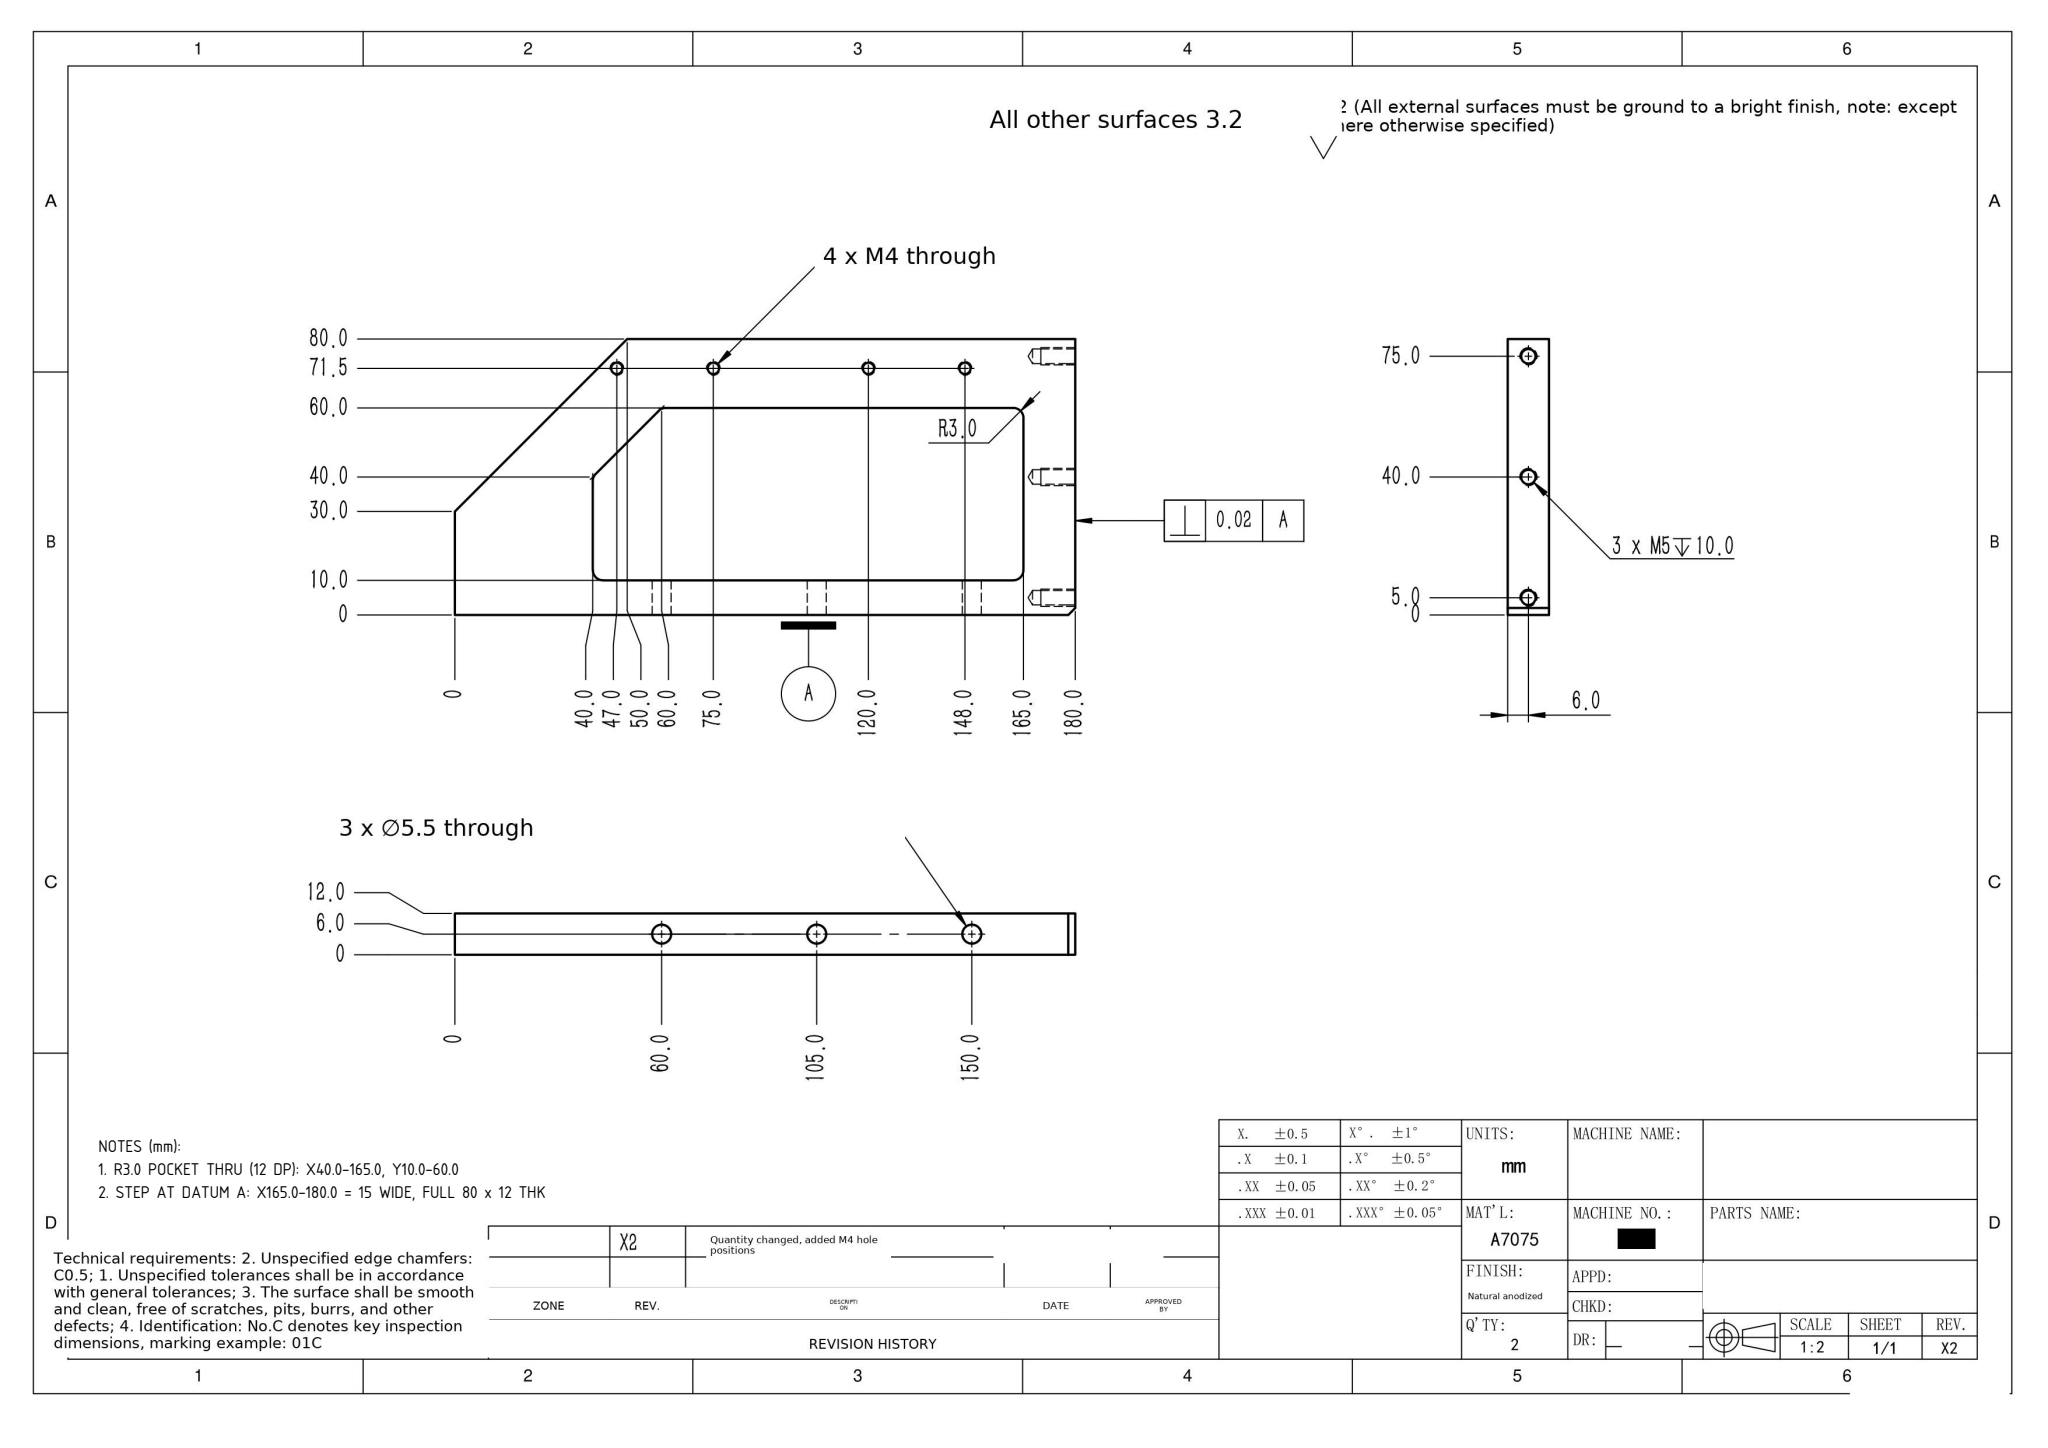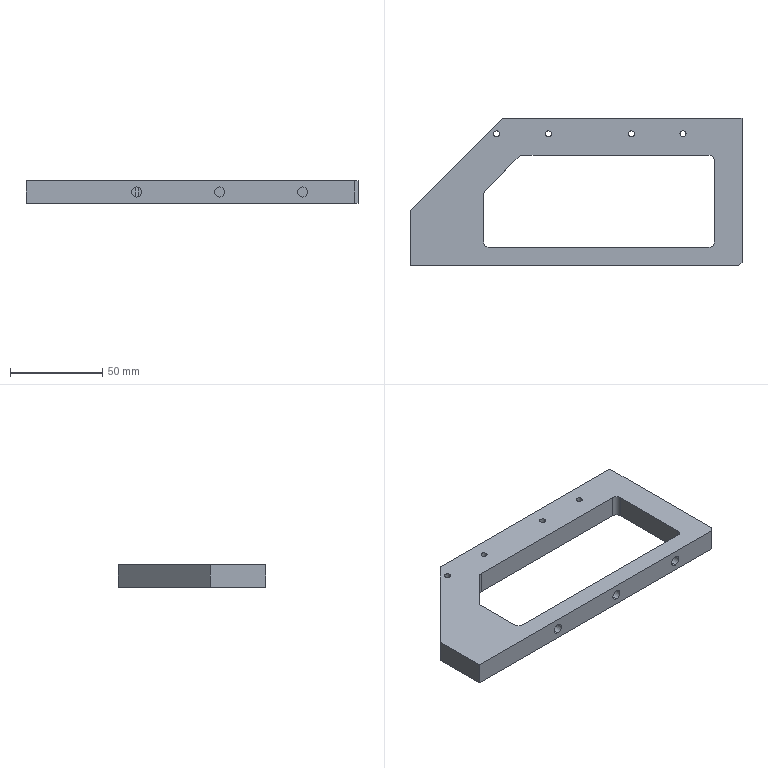Part | SolidWorks | mm | 1 solid | 44 faces | box 180 x 80 x 12 mm | volume 83594 mm3 | cylinder 25 | plane 13 | cone 6 | commonest cylinder face diameters 3.3 x8 4.2 x6 5.5 x6 6 x5
Drawing notes:
R3.0 POCKET THRU (12 DP): X40.0-165.0, Y10.0-60.0 | from the solid: Ø6.0 (R3.0) corner cyls at (43,13),(43,38.76),(61.24,57),(162,13),(162,57), len 12.0 = full thk; planes x=40/165, y=10/60
STEP AT DATUM A: X165.0-180.0 = 15 WIDE, FULL 80 x 12 THK | from the solid: axis planes x=165.0 and x=180.0; bbox 180x80x12; M5 holes (Ø4.2, x-axis) at z=6.0 enter from x=180 face
build123d program:
from build123d import *

# Parameters (mm, degrees)
SKETCH1_W             = 180
SKETCH1_H             = 80
BOSS_EXTRUDE1_DEPTH   = 6
CHAMFER1_SIZE         = 50
SKETCH2_W             = 125
SKETCH2_H             = 50
CUT_EXTRUDE1_DEPTH    = 100.217
CHAMFER2_SIZE         = 20
SKETCH3_R             = 2.75
CUT_EXTRUDE2_DEPTH    = 10
LPATTERN1_COUNT       = 3
LPATTERN1_PITCH       = 45
M5_TAPPED_HOLE1_D     = 4.2
M5_TAPPED_HOLE1_DEPTH = 12.4
M5_TAPPED_HOLE1_TIP   = 1.262
FILLET1_R             = 3
CHAMFER3_SIZE         = 2
M4_TAPPED_HOLE1_D     = 3.3


with BuildPart() as part:
    # Sketch1 → Boss-Extrude1 (new, symmetric)
    with BuildSketch(Plane.XY):
        Rectangle(SKETCH1_W, SKETCH1_H)
    extrude(amount=BOSS_EXTRUDE1_DEPTH, both=True)

    # Chamfer1
    chamfer1_edges = [part.edges().sort_by_distance(p)[0] for p in [
        (-90, 40, 0),
    ]]
    chamfer(chamfer1_edges, length=CHAMFER1_SIZE)

    # Sketch2 → Cut-Extrude1 (cut, through all)
    with BuildSketch(Plane.XY.offset(6)):
        with Locations((12.5, -5)):
            Rectangle(SKETCH2_W, SKETCH2_H)
    extrude(amount=-CUT_EXTRUDE1_DEPTH, mode=Mode.SUBTRACT)

    # Chamfer2
    chamfer2_edges = [part.edges().sort_by_distance(p)[0] for p in [
        (-50, 20, 0),
    ]]
    chamfer(chamfer2_edges, length=CHAMFER2_SIZE)

    # Sketch3 → Cut-Extrude2 (cut)
    with BuildSketch(Plane.XZ.offset(40)):
        with Locations(Location((60, 0, 0), (0, 0, 270))):
            Circle(SKETCH3_R)
    cut_extrude2 = extrude(amount=-CUT_EXTRUDE2_DEPTH, mode=Mode.SUBTRACT)

    # LPattern1: Cut-Extrude2 ×3
    with Locations(*[(-i * LPATTERN1_PITCH, 0, 0) for i in range(1, LPATTERN1_COUNT)]):
        add(cut_extrude2, mode=Mode.SUBTRACT)

    # M5 Tapped Hole1
    with Locations(Plane(origin=(90, 0, 0), x_dir=(0, 0, -1), z_dir=(1, 0, 0))):
        with Locations((0, 35), (0, 0), (0, -35)):
            Hole(M5_TAPPED_HOLE1_D / 2, depth=M5_TAPPED_HOLE1_DEPTH)
            with Locations((0, 0, -(M5_TAPPED_HOLE1_DEPTH + M5_TAPPED_HOLE1_TIP / 2))):  # 118° drill point
                Cone(0, M5_TAPPED_HOLE1_D / 2, M5_TAPPED_HOLE1_TIP, mode=Mode.SUBTRACT)

    # Fillet1
    fillet1_edges = [part.edges().sort_by_distance(p)[0] for p in [
        (-50, -30, 0),
        (75, 20, 0),
        (75, -30, 0),
        (-50, 0, 0),
        (-30, 20, 0),
    ]]
    fillet(fillet1_edges, radius=FILLET1_R)

    # Chamfer3
    chamfer3_edges = [part.edges().sort_by_distance(p)[0] for p in [
        (90, -40, 0),
    ]]
    chamfer(chamfer3_edges, length=CHAMFER3_SIZE)

    # M4 Tapped Hole1 (through all)
    with Locations(Plane(origin=(0, 0, -6), x_dir=(-1, 0, 0), z_dir=(0, 0, -1))):
        with Locations((-58, 31.5), (-30, 31.5), (15, 31.5), (43, 31.5)):
            Hole(M4_TAPPED_HOLE1_D / 2)


solid = part.part